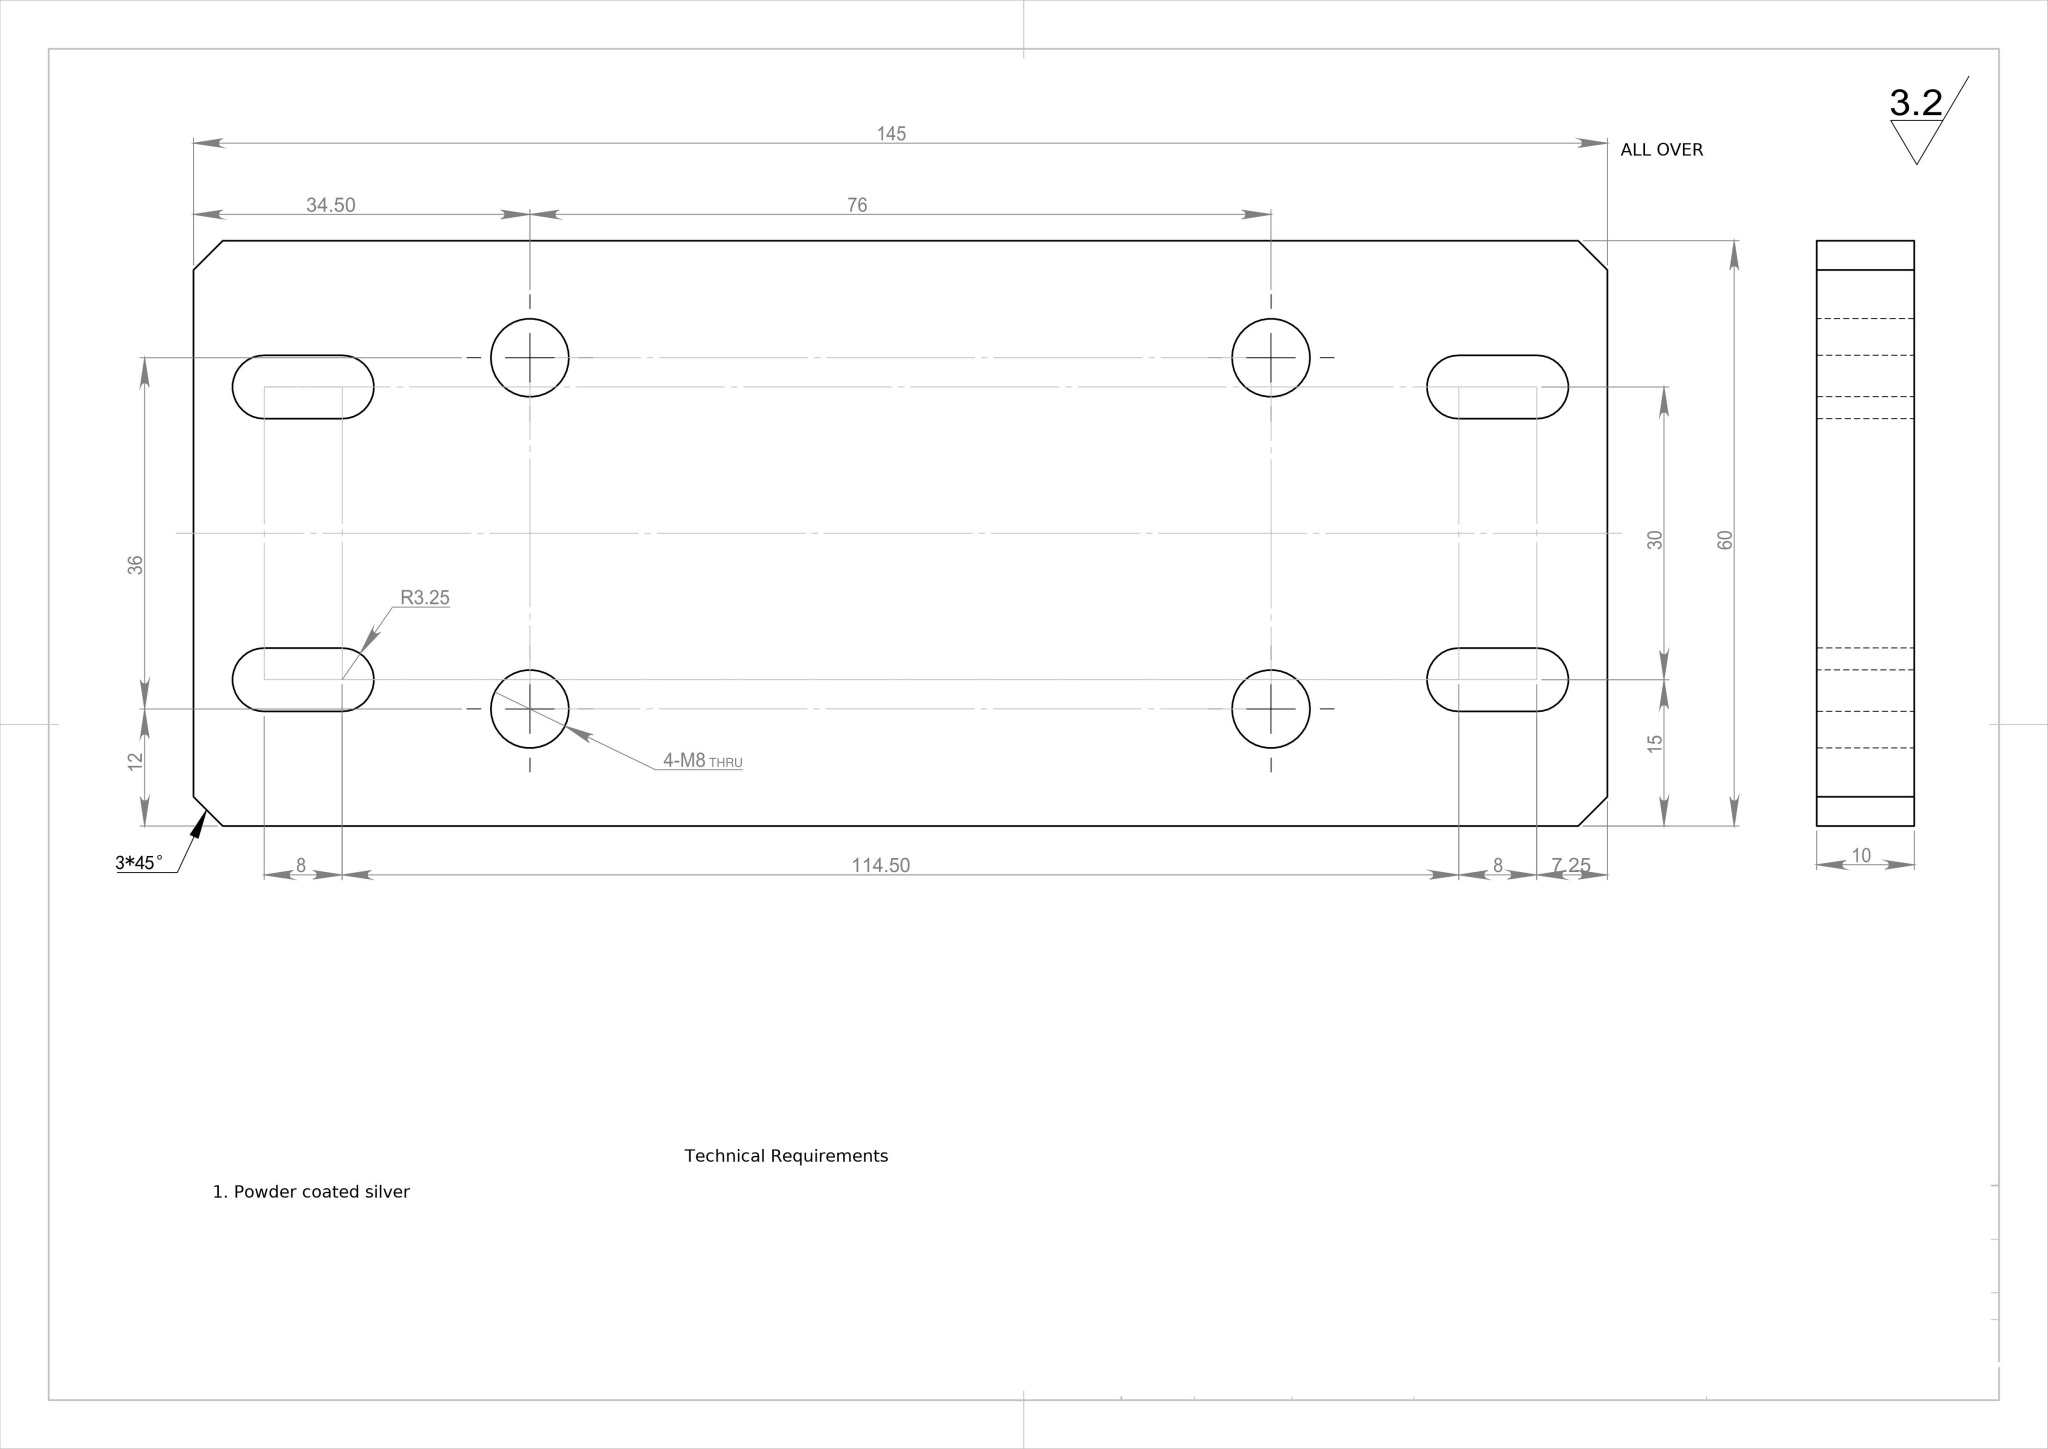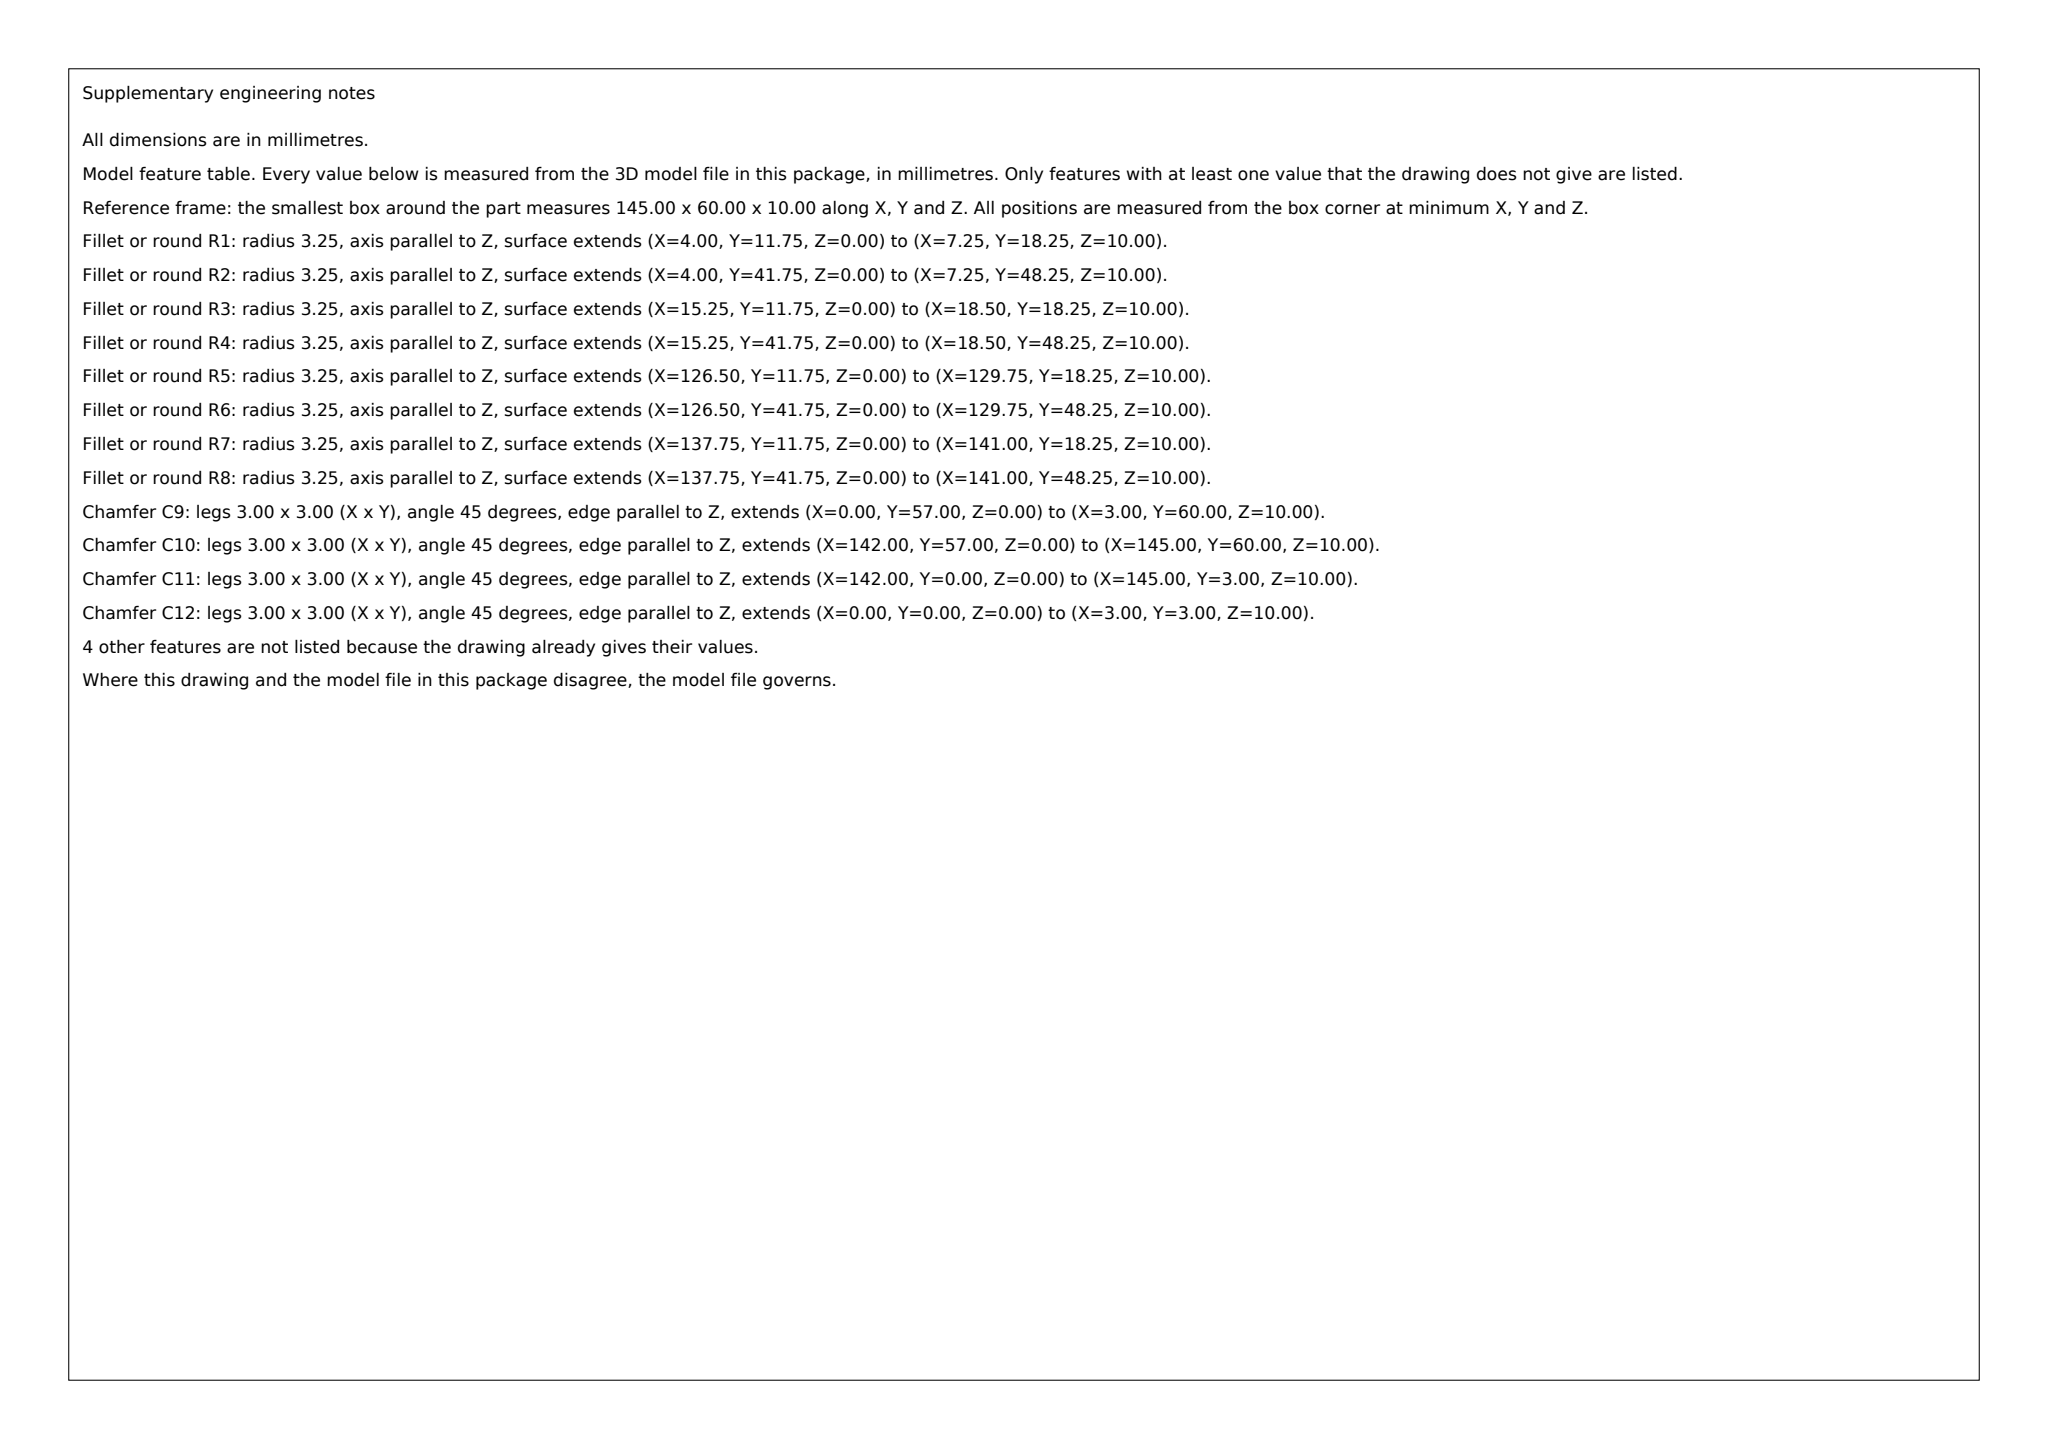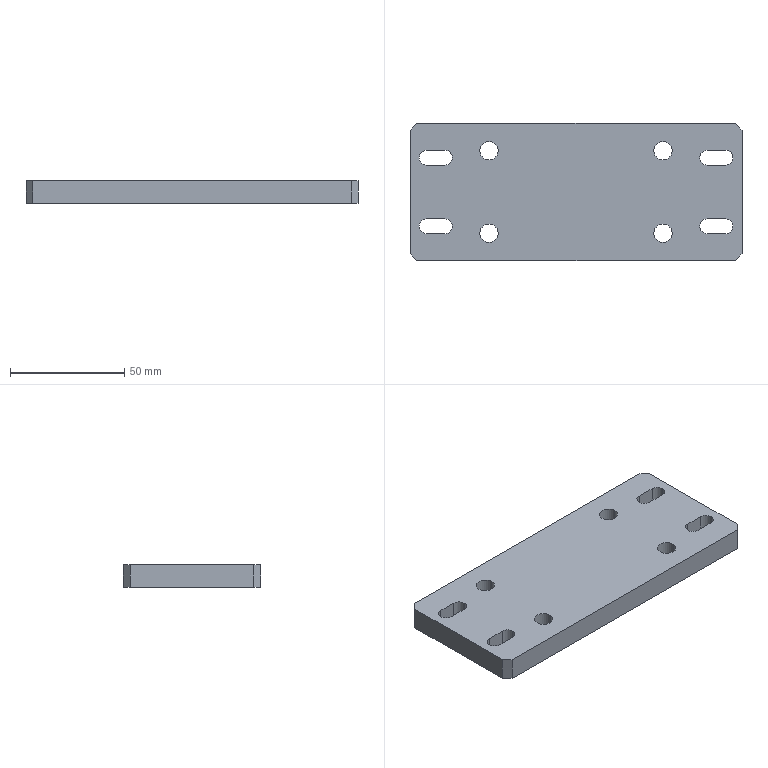Part | SolidWorks | mm | 1 solid | 38 faces | box 145 x 60 x 10 mm | volume 81402 mm3 | cylinder 20 | plane 18 | commonest cylinder face diameters 6.5 x12 8 x8
build123d program:
from build123d import *

# Parameters (mm, degrees)
SKETCH1_W               = 145
SKETCH1_H               = 60
BOSS_EXTRUDE1_DEPTH     = 10
CHAMFER1_SIZE           = 3
CUT_EXTRUDE4_DEPTH      = 80.096
MIRROR3_COPY_1_DEPTH    = 80.096
SKETCH6_R               = 4
CUT_EXTRUDE5_DEPTH      = 80.096
MIRROR5_COPY_1_SKETCH_R = 4
MIRROR5_COPY_1_DEPTH    = 80.096


with BuildPart() as part:
    # Sketch1 → Boss-Extrude1 (new body)
    with BuildSketch(Plane.XY):
        Rectangle(SKETCH1_W, SKETCH1_H)
    extrude(amount=BOSS_EXTRUDE1_DEPTH)

    # Chamfer1
    chamfer1_edges = [part.edges().sort_by_distance(p)[0] for p in [
        (72.5, -30, 5),
        (-72.5, -30, 5),
        (-72.5, 30, 5),
        (72.5, 30, 5),
    ]]
    chamfer(chamfer1_edges, length=CHAMFER1_SIZE)

    # Sketch5 → Cut-Extrude4 (cut, through all)
    with BuildSketch(Plane.XY.offset(10)):
        with BuildLine():
            Line((57.25, 18.25), (65.25, 18.25))
            ThreePointArc((65.25, 18.25), (68.5, 15), (65.25, 11.75))
            Line((65.25, 11.75), (57.25, 11.75))
            ThreePointArc((57.25, 11.75), (54, 15), (57.25, 18.25))
        make_face()
    cut_extrude4 = extrude(amount=-CUT_EXTRUDE4_DEPTH, mode=Mode.SUBTRACT)

    # Mirror2: Cut-Extrude4 across plane
    add(cut_extrude4.mirror(Plane(origin=(0, 0, 0), x_dir=(0, 0, 1), z_dir=(1, 0, 0))), mode=Mode.SUBTRACT)

    # Mirror3: Cut-Extrude4 across plane
    add(cut_extrude4.mirror(Plane.ZX), mode=Mode.SUBTRACT)

    # Mirror3 copy 1 sketch → Mirror3 copy 1 (cut, through all)
    with BuildSketch(Plane(origin=(0, 0, 10), x_dir=(-1, 0, 0), z_dir=(0, 0, 1))):
        with BuildLine():
            Line((57.25, 18.25), (65.25, 18.25))
            ThreePointArc((65.25, 18.25), (68.5, 15), (65.25, 11.75))
            Line((65.25, 11.75), (57.25, 11.75))
            ThreePointArc((57.25, 11.75), (54, 15), (57.25, 18.25))
        make_face()
    extrude(amount=-MIRROR3_COPY_1_DEPTH, mode=Mode.SUBTRACT)

    # Sketch6 → Cut-Extrude5 (cut, through all)
    with BuildSketch(Plane.XY.offset(10)):
        with Locations((-38, 18)):
            Circle(SKETCH6_R)
    cut_extrude5 = extrude(amount=-CUT_EXTRUDE5_DEPTH, mode=Mode.SUBTRACT)

    # Mirror4: Cut-Extrude5 across plane
    add(cut_extrude5.mirror(Plane(origin=(0, 0, 0), x_dir=(0, 0, 1), z_dir=(1, 0, 0))), mode=Mode.SUBTRACT)

    # Mirror5: Cut-Extrude5 across plane
    add(cut_extrude5.mirror(Plane.ZX), mode=Mode.SUBTRACT)

    # Mirror5 copy 1 sketch → Mirror5 copy 1 (cut, through all)
    with BuildSketch(Plane(origin=(0, 0, 10), x_dir=(-1, 0, 0), z_dir=(0, 0, 1))):
        with Locations((-38, 18)):
            Circle(MIRROR5_COPY_1_SKETCH_R)
    extrude(amount=-MIRROR5_COPY_1_DEPTH, mode=Mode.SUBTRACT)


solid = part.part